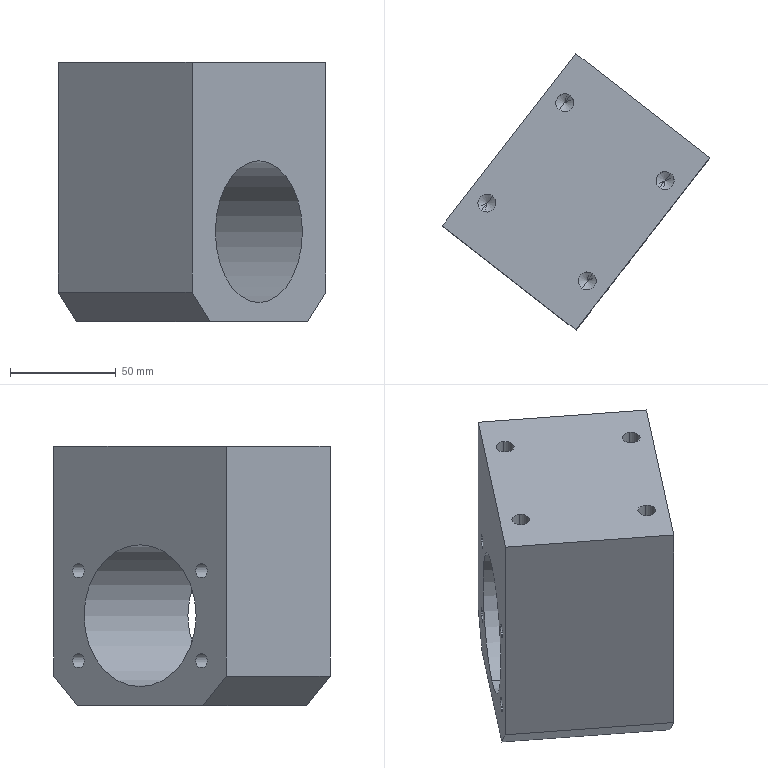Component | SolidWorks | 0803_206_Holder-1 | 1 solid | 42 faces | box 126.35 x 130.42 x 122.5 mm | volume 700208 mm3 | cylinder 18 | cone 16 | plane 8 | commonest cylinder face diameters 8.5 x8 6.8 x8 67 x2
STEP:
#1=COLOUR_RGB('',0.7922,0.8196,0.9333);
#2=FILL_AREA_STYLE_COLOUR('',#1);
#3=FILL_AREA_STYLE('',(#2));
#4=SURFACE_STYLE_FILL_AREA(#3);
#5=SURFACE_SIDE_STYLE('',(#4));
#6=SURFACE_STYLE_USAGE(.BOTH.,#5);
#7=PRESENTATION_STYLE_ASSIGNMENT((#6));
#8=CARTESIAN_POINT('',(2.329,25.802,12.851));
#9=VERTEX_POINT('',#8);
#10=CARTESIAN_POINT('',(2.534,26.066,12.851));
#11=VERTEX_POINT('',#10);
#12=CARTESIAN_POINT('',(2.431,25.934,12.851));
#13=DIRECTION('',(-0.,-0.,1.));
#14=DIRECTION('',(0.6132,0.7899,0.));
#15=AXIS2_PLACEMENT_3D('',#12,#13,#14);
#16=CIRCLE('',#15,0.1673);
#17=EDGE_CURVE('',#9,#11,#16,.T.);
#18=ORIENTED_EDGE('',*,*,#17,.F.);
#19=CARTESIAN_POINT('',(2.329,25.802,14.032));
#20=VERTEX_POINT('',#19);
#21=CARTESIAN_POINT('',(2.329,25.802,14.032));
#22=DIRECTION('',(-0.,-0.,1.));
#23=VECTOR('',#22,39.37);
#24=LINE('',#21,#23);
#25=EDGE_CURVE('',#9,#20,#24,.T.);
#26=ORIENTED_EDGE('',*,*,#25,.T.);
#27=CARTESIAN_POINT('',(2.534,26.066,14.032));
#28=VERTEX_POINT('',#27);
#29=CARTESIAN_POINT('',(2.431,25.934,14.032));
#30=DIRECTION('',(-0.,-0.,1.));
#31=DIRECTION('',(0.6132,0.7899,0.));
#32=AXIS2_PLACEMENT_3D('',#29,#30,#31);
#33=CIRCLE('',#32,0.1673);
#34=EDGE_CURVE('',#20,#28,#33,.T.);
#35=ORIENTED_EDGE('',*,*,#34,.T.);
#36=CARTESIAN_POINT('',(2.534,26.066,14.032));
#37=DIRECTION('',(-0.,-0.,1.));
#38=VECTOR('',#37,39.37);
#39=LINE('',#36,#38);
#40=EDGE_CURVE('',#11,#28,#39,.T.);
#41=ORIENTED_EDGE('',*,*,#40,.F.);
#42=EDGE_LOOP('',(#18,#26,#35,#41));
#43=FACE_OUTER_BOUND('',#42,.T.);
#44=CARTESIAN_POINT('',(2.431,25.934,14.032));
#45=DIRECTION('',(-0.,-0.,1.));
#46=DIRECTION('',(0.6132,0.7899,0.));
#47=AXIS2_PLACEMENT_3D('',#44,#45,#46);
#48=CYLINDRICAL_SURFACE('',#47,0.1673);
#49=ADVANCED_FACE('',(#43),#48,.F.);
#50=CARTESIAN_POINT('',(2.431,25.934,12.75));
#51=VERTEX_POINT('',#50);
#52=CARTESIAN_POINT('',(2.534,26.066,12.851));
#53=DIRECTION('',(0.5256,0.6771,0.515));
#54=VECTOR('',#53,39.37);
#55=LINE('',#52,#54);
#56=EDGE_CURVE('',#51,#11,#55,.T.);
#57=ORIENTED_EDGE('',*,*,#56,.F.);
#58=CARTESIAN_POINT('',(2.329,25.802,12.851));
#59=DIRECTION('',(-0.5256,-0.6771,0.515));
#60=VECTOR('',#59,39.37);
#61=LINE('',#58,#60);
#62=EDGE_CURVE('',#51,#9,#61,.T.);
#63=ORIENTED_EDGE('',*,*,#62,.T.);
#64=ORIENTED_EDGE('',*,*,#17,.T.);
#65=EDGE_LOOP('',(#57,#63,#64));
#66=FACE_OUTER_BOUND('',#65,.T.);
#67=CARTESIAN_POINT('',(2.431,25.934,12.851));
#68=DIRECTION('',(-0.,-0.,1.));
#69=DIRECTION('',(0.6132,0.7899,0.));
#70=AXIS2_PLACEMENT_3D('',#67,#68,#69);
#71=CONICAL_SURFACE('',#70,0.1673,1.03);
#72=ADVANCED_FACE('',(#66),#71,.F.);
#73=CARTESIAN_POINT('',(4.195,24.353,12.851));
#74=VERTEX_POINT('',#73);
#75=CARTESIAN_POINT('',(4.4,24.618,12.851));
#76=VERTEX_POINT('',#75);
#77=CARTESIAN_POINT('',(4.297,24.486,12.851));
#78=DIRECTION('',(-0.,-0.,1.));
#79=DIRECTION('',(0.6132,0.7899,0.));
#80=AXIS2_PLACEMENT_3D('',#77,#78,#79);
#81=CIRCLE('',#80,0.1673);
#82=EDGE_CURVE('',#74,#76,#81,.T.);
#83=ORIENTED_EDGE('',*,*,#82,.F.);
#84=CARTESIAN_POINT('',(4.195,24.353,14.032));
#85=VERTEX_POINT('',#84);
#86=CARTESIAN_POINT('',(4.195,24.353,14.032));
#87=DIRECTION('',(-0.,-0.,1.));
#88=VECTOR('',#87,39.37);
#89=LINE('',#86,#88);
#90=EDGE_CURVE('',#74,#85,#89,.T.);
#91=ORIENTED_EDGE('',*,*,#90,.T.);
#92=CARTESIAN_POINT('',(4.4,24.618,14.032));
#93=VERTEX_POINT('',#92);
#94=CARTESIAN_POINT('',(4.297,24.486,14.032));
#95=DIRECTION('',(-0.,-0.,1.));
#96=DIRECTION('',(0.6132,0.7899,0.));
#97=AXIS2_PLACEMENT_3D('',#94,#95,#96);
#98=CIRCLE('',#97,0.1673);
#99=EDGE_CURVE('',#85,#93,#98,.T.);
#100=ORIENTED_EDGE('',*,*,#99,.T.);
#101=CARTESIAN_POINT('',(4.4,24.618,14.032));
#102=DIRECTION('',(-0.,-0.,1.));
#103=VECTOR('',#102,39.37);
#104=LINE('',#101,#103);
#105=EDGE_CURVE('',#76,#93,#104,.T.);
#106=ORIENTED_EDGE('',*,*,#105,.F.);
#107=EDGE_LOOP('',(#83,#91,#100,#106));
#108=FACE_OUTER_BOUND('',#107,.T.);
#109=CARTESIAN_POINT('',(4.297,24.486,14.032));
#110=DIRECTION('',(-0.,-0.,1.));
#111=DIRECTION('',(0.6132,0.7899,0.));
#112=AXIS2_PLACEMENT_3D('',#109,#110,#111);
#113=CYLINDRICAL_SURFACE('',#112,0.1673);
#114=ADVANCED_FACE('',(#108),#113,.F.);
#115=CARTESIAN_POINT('',(4.297,24.486,12.75));
#116=VERTEX_POINT('',#115);
#117=CARTESIAN_POINT('',(4.4,24.618,12.851));
#118=DIRECTION('',(0.5256,0.6771,0.515));
#119=VECTOR('',#118,39.37);
#120=LINE('',#117,#119);
#121=EDGE_CURVE('',#116,#76,#120,.T.);
#122=ORIENTED_EDGE('',*,*,#121,.F.);
#123=CARTESIAN_POINT('',(4.195,24.353,12.851));
#124=DIRECTION('',(-0.5256,-0.6771,0.515));
#125=VECTOR('',#124,39.37);
#126=LINE('',#123,#125);
#127=EDGE_CURVE('',#116,#74,#126,.T.);
#128=ORIENTED_EDGE('',*,*,#127,.T.);
#129=ORIENTED_EDGE('',*,*,#82,.T.);
#130=EDGE_LOOP('',(#122,#128,#129));
#131=FACE_OUTER_BOUND('',#130,.T.);
#132=CARTESIAN_POINT('',(4.297,24.486,12.851));
#133=DIRECTION('',(-0.,-0.,1.));
#134=DIRECTION('',(0.6132,0.7899,0.));
#135=AXIS2_PLACEMENT_3D('',#132,#133,#134);
#136=CONICAL_SURFACE('',#135,0.1673,1.03);
#137=ADVANCED_FACE('',(#131),#136,.F.);
#138=CARTESIAN_POINT('',(5.643,26.219,12.851));
#139=VERTEX_POINT('',#138);
#140=CARTESIAN_POINT('',(5.848,26.484,12.851));
#141=VERTEX_POINT('',#140);
#142=CARTESIAN_POINT('',(5.746,26.352,12.851));
#143=DIRECTION('',(-0.,-0.,1.));
#144=DIRECTION('',(0.6132,0.7899,0.));
#145=AXIS2_PLACEMENT_3D('',#142,#143,#144);
#146=CIRCLE('',#145,0.1673);
#147=EDGE_CURVE('',#139,#141,#146,.T.);
#148=ORIENTED_EDGE('',*,*,#147,.F.);
#149=CARTESIAN_POINT('',(5.643,26.219,14.032));
#150=VERTEX_POINT('',#149);
#151=CARTESIAN_POINT('',(5.643,26.219,14.032));
#152=DIRECTION('',(-0.,-0.,1.));
#153=VECTOR('',#152,39.37);
#154=LINE('',#151,#153);
#155=EDGE_CURVE('',#139,#150,#154,.T.);
#156=ORIENTED_EDGE('',*,*,#155,.T.);
#157=CARTESIAN_POINT('',(5.848,26.484,14.032));
#158=VERTEX_POINT('',#157);
#159=CARTESIAN_POINT('',(5.746,26.352,14.032));
#160=DIRECTION('',(-0.,-0.,1.));
#161=DIRECTION('',(0.6132,0.7899,0.));
#162=AXIS2_PLACEMENT_3D('',#159,#160,#161);
#163=CIRCLE('',#162,0.1673);
#164=EDGE_CURVE('',#150,#158,#163,.T.);
#165=ORIENTED_EDGE('',*,*,#164,.T.);
#166=CARTESIAN_POINT('',(5.848,26.484,14.032));
#167=DIRECTION('',(-0.,-0.,1.));
#168=VECTOR('',#167,39.37);
#169=LINE('',#166,#168);
#170=EDGE_CURVE('',#141,#158,#169,.T.);
#171=ORIENTED_EDGE('',*,*,#170,.F.);
#172=EDGE_LOOP('',(#148,#156,#165,#171));
#173=FACE_OUTER_BOUND('',#172,.T.);
#174=CARTESIAN_POINT('',(5.746,26.352,14.032));
#175=DIRECTION('',(-0.,-0.,1.));
#176=DIRECTION('',(0.6132,0.7899,0.));
#177=AXIS2_PLACEMENT_3D('',#174,#175,#176);
#178=CYLINDRICAL_SURFACE('',#177,0.1673);
#179=ADVANCED_FACE('',(#173),#178,.F.);
#180=CARTESIAN_POINT('',(5.746,26.352,12.75));
#181=VERTEX_POINT('',#180);
#182=CARTESIAN_POINT('',(5.848,26.484,12.851));
#183=DIRECTION('',(0.5256,0.6771,0.515));
#184=VECTOR('',#183,39.37);
#185=LINE('',#182,#184);
#186=EDGE_CURVE('',#181,#141,#185,.T.);
#187=ORIENTED_EDGE('',*,*,#186,.F.);
#188=CARTESIAN_POINT('',(5.643,26.219,12.851));
#189=DIRECTION('',(-0.5256,-0.6771,0.515));
#190=VECTOR('',#189,39.37);
#191=LINE('',#188,#190);
#192=EDGE_CURVE('',#181,#139,#191,.T.);
#193=ORIENTED_EDGE('',*,*,#192,.T.);
#194=ORIENTED_EDGE('',*,*,#147,.T.);
#195=EDGE_LOOP('',(#187,#193,#194));
#196=FACE_OUTER_BOUND('',#195,.T.);
#197=CARTESIAN_POINT('',(5.746,26.352,12.851));
#198=DIRECTION('',(-0.,-0.,1.));
#199=DIRECTION('',(0.6132,0.7899,0.));
#200=AXIS2_PLACEMENT_3D('',#197,#198,#199);
#201=CONICAL_SURFACE('',#200,0.1673,1.03);
#202=ADVANCED_FACE('',(#196),#201,.F.);
#203=CARTESIAN_POINT('',(3.777,27.668,12.851));
#204=VERTEX_POINT('',#203);
#205=CARTESIAN_POINT('',(3.982,27.932,12.851));
#206=VERTEX_POINT('',#205);
#207=CARTESIAN_POINT('',(3.88,27.8,12.851));
#208=DIRECTION('',(-0.,-0.,1.));
#209=DIRECTION('',(0.6132,0.7899,0.));
#210=AXIS2_PLACEMENT_3D('',#207,#208,#209);
#211=CIRCLE('',#210,0.1673);
#212=EDGE_CURVE('',#204,#206,#211,.T.);
#213=ORIENTED_EDGE('',*,*,#212,.F.);
#214=CARTESIAN_POINT('',(3.777,27.668,14.032));
#215=VERTEX_POINT('',#214);
#216=CARTESIAN_POINT('',(3.777,27.668,14.032));
#217=DIRECTION('',(-0.,-0.,1.));
#218=VECTOR('',#217,39.37);
#219=LINE('',#216,#218);
#220=EDGE_CURVE('',#204,#215,#219,.T.);
#221=ORIENTED_EDGE('',*,*,#220,.T.);
#222=CARTESIAN_POINT('',(3.982,27.932,14.032));
#223=VERTEX_POINT('',#222);
#224=CARTESIAN_POINT('',(3.88,27.8,14.032));
#225=DIRECTION('',(-0.,-0.,1.));
#226=DIRECTION('',(0.6132,0.7899,0.));
#227=AXIS2_PLACEMENT_3D('',#224,#225,#226);
#228=CIRCLE('',#227,0.1673);
#229=EDGE_CURVE('',#215,#223,#228,.T.);
#230=ORIENTED_EDGE('',*,*,#229,.T.);
#231=CARTESIAN_POINT('',(3.982,27.932,14.032));
#232=DIRECTION('',(-0.,-0.,1.));
#233=VECTOR('',#232,39.37);
#234=LINE('',#231,#233);
#235=EDGE_CURVE('',#206,#223,#234,.T.);
#236=ORIENTED_EDGE('',*,*,#235,.F.);
#237=EDGE_LOOP('',(#213,#221,#230,#236));
#238=FACE_OUTER_BOUND('',#237,.T.);
#239=CARTESIAN_POINT('',(3.88,27.8,14.032));
#240=DIRECTION('',(-0.,-0.,1.));
#241=DIRECTION('',(0.6132,0.7899,0.));
#242=AXIS2_PLACEMENT_3D('',#239,#240,#241);
#243=CYLINDRICAL_SURFACE('',#242,0.1673);
#244=ADVANCED_FACE('',(#238),#243,.F.);
#245=CARTESIAN_POINT('',(3.88,27.8,12.75));
#246=VERTEX_POINT('',#245);
#247=CARTESIAN_POINT('',(3.982,27.932,12.851));
#248=DIRECTION('',(0.5256,0.6771,0.515));
#249=VECTOR('',#248,39.37);
#250=LINE('',#247,#249);
#251=EDGE_CURVE('',#246,#206,#250,.T.);
#252=ORIENTED_EDGE('',*,*,#251,.F.);
#253=CARTESIAN_POINT('',(3.777,27.668,12.851));
#254=DIRECTION('',(-0.5256,-0.6771,0.515));
#255=VECTOR('',#254,39.37);
#256=LINE('',#253,#255);
#257=EDGE_CURVE('',#246,#204,#256,.T.);
#258=ORIENTED_EDGE('',*,*,#257,.T.);
#259=ORIENTED_EDGE('',*,*,#212,.T.);
#260=EDGE_LOOP('',(#252,#258,#259));
#261=FACE_OUTER_BOUND('',#260,.T.);
#262=CARTESIAN_POINT('',(3.88,27.8,12.851));
#263=DIRECTION('',(-0.,-0.,1.));
#264=DIRECTION('',(0.6132,0.7899,0.));
#265=AXIS2_PLACEMENT_3D('',#262,#263,#264);
#266=CONICAL_SURFACE('',#265,0.1673,1.03);
#267=ADVANCED_FACE('',(#261),#266,.F.);
#268=CARTESIAN_POINT('',(4.666,27.529,11.585));
#269=VERTEX_POINT('',#268);
#270=CARTESIAN_POINT('',(4.666,27.529,11.853));
#271=VERTEX_POINT('',#270);
#272=CARTESIAN_POINT('',(4.666,27.529,11.719));
#273=DIRECTION('',(-0.7899,0.6132,0.));
#274=DIRECTION('',(0.,0.,1.));
#275=AXIS2_PLACEMENT_3D('',#272,#273,#274);
#276=CIRCLE('',#275,0.1339);
#277=EDGE_CURVE('',#269,#271,#276,.T.);
#278=ORIENTED_EDGE('',*,*,#277,.F.);
#279=CARTESIAN_POINT('',(3.733,28.253,11.585));
#280=VERTEX_POINT('',#279);
#281=CARTESIAN_POINT('',(3.733,28.253,11.585));
#282=DIRECTION('',(-0.7899,0.6132,0.));
#283=VECTOR('',#282,39.37);
#284=LINE('',#281,#283);
#285=EDGE_CURVE('',#269,#280,#284,.T.);
#286=ORIENTED_EDGE('',*,*,#285,.T.);
#287=CARTESIAN_POINT('',(3.733,28.253,11.853));
#288=VERTEX_POINT('',#287);
#289=CARTESIAN_POINT('',(3.733,28.253,11.719));
#290=DIRECTION('',(-0.7899,0.6132,0.));
#291=DIRECTION('',(0.,0.,1.));
#292=AXIS2_PLACEMENT_3D('',#289,#290,#291);
#293=CIRCLE('',#292,0.1339);
#294=EDGE_CURVE('',#280,#288,#293,.T.);
#295=ORIENTED_EDGE('',*,*,#294,.T.);
#296=CARTESIAN_POINT('',(3.733,28.253,11.853));
#297=DIRECTION('',(-0.7899,0.6132,0.));
#298=VECTOR('',#297,39.37);
#299=LINE('',#296,#298);
#300=EDGE_CURVE('',#271,#288,#299,.T.);
#301=ORIENTED_EDGE('',*,*,#300,.F.);
#302=EDGE_LOOP('',(#278,#286,#295,#301));
#303=FACE_OUTER_BOUND('',#302,.T.);
#304=CARTESIAN_POINT('',(3.733,28.253,11.719));
#305=DIRECTION('',(-0.7899,0.6132,0.));
#306=DIRECTION('',(0.,0.,1.));
#307=AXIS2_PLACEMENT_3D('',#304,#305,#306);
#308=CYLINDRICAL_SURFACE('',#307,0.1339);
#309=ADVANCED_FACE('',(#303),#308,.F.);
#310=CARTESIAN_POINT('',(4.73,27.48,11.719));
#311=VERTEX_POINT('',#310);
#312=CARTESIAN_POINT('',(4.666,27.529,11.853));
#313=DIRECTION('',(-0.4068,0.3158,0.8572));
#314=VECTOR('',#313,39.37);
#315=LINE('',#312,#314);
#316=EDGE_CURVE('',#311,#271,#315,.T.);
#317=ORIENTED_EDGE('',*,*,#316,.F.);
#318=CARTESIAN_POINT('',(4.666,27.529,11.585));
#319=DIRECTION('',(-0.4068,0.3158,-0.8572));
#320=VECTOR('',#319,39.37);
#321=LINE('',#318,#320);
#322=EDGE_CURVE('',#311,#269,#321,.T.);
#323=ORIENTED_EDGE('',*,*,#322,.T.);
#324=ORIENTED_EDGE('',*,*,#277,.T.);
#325=EDGE_LOOP('',(#317,#323,#324));
#326=FACE_OUTER_BOUND('',#325,.T.);
#327=CARTESIAN_POINT('',(4.666,27.529,11.719));
#328=DIRECTION('',(-0.7899,0.6132,0.));
#329=DIRECTION('',(0.,0.,1.));
#330=AXIS2_PLACEMENT_3D('',#327,#328,#329);
#331=CONICAL_SURFACE('',#330,0.1339,1.03);
#332=ADVANCED_FACE('',(#326),#331,.F.);
#333=CARTESIAN_POINT('',(4.666,27.529,9.912));
#334=VERTEX_POINT('',#333);
#335=CARTESIAN_POINT('',(4.666,27.529,10.18));
#336=VERTEX_POINT('',#335);
#337=CARTESIAN_POINT('',(4.666,27.529,10.046));
#338=DIRECTION('',(-0.7899,0.6132,0.));
#339=DIRECTION('',(0.,0.,1.));
#340=AXIS2_PLACEMENT_3D('',#337,#338,#339);
#341=CIRCLE('',#340,0.1339);
#342=EDGE_CURVE('',#334,#336,#341,.T.);
#343=ORIENTED_EDGE('',*,*,#342,.F.);
#344=CARTESIAN_POINT('',(3.733,28.253,9.912));
#345=VERTEX_POINT('',#344);
#346=CARTESIAN_POINT('',(3.733,28.253,9.912));
#347=DIRECTION('',(-0.7899,0.6132,0.));
#348=VECTOR('',#347,39.37);
#349=LINE('',#346,#348);
#350=EDGE_CURVE('',#334,#345,#349,.T.);
#351=ORIENTED_EDGE('',*,*,#350,.T.);
#352=CARTESIAN_POINT('',(3.733,28.253,10.18));
#353=VERTEX_POINT('',#352);
#354=CARTESIAN_POINT('',(3.733,28.253,10.046));
#355=DIRECTION('',(-0.7899,0.6132,0.));
#356=DIRECTION('',(0.,0.,1.));
#357=AXIS2_PLACEMENT_3D('',#354,#355,#356);
#358=CIRCLE('',#357,0.1339);
#359=EDGE_CURVE('',#345,#353,#358,.T.);
#360=ORIENTED_EDGE('',*,*,#359,.T.);
#361=CARTESIAN_POINT('',(3.733,28.253,10.18));
#362=DIRECTION('',(-0.7899,0.6132,0.));
#363=VECTOR('',#362,39.37);
#364=LINE('',#361,#363);
#365=EDGE_CURVE('',#336,#353,#364,.T.);
#366=ORIENTED_EDGE('',*,*,#365,.F.);
#367=EDGE_LOOP('',(#343,#351,#360,#366));
#368=FACE_OUTER_BOUND('',#367,.T.);
#369=CARTESIAN_POINT('',(3.733,28.253,10.046));
#370=DIRECTION('',(-0.7899,0.6132,0.));
#371=DIRECTION('',(0.,0.,1.));
#372=AXIS2_PLACEMENT_3D('',#369,#370,#371);
#373=CYLINDRICAL_SURFACE('',#372,0.1339);
#374=ADVANCED_FACE('',(#368),#373,.F.);
#375=CARTESIAN_POINT('',(4.73,27.48,10.046));
#376=VERTEX_POINT('',#375);
#377=CARTESIAN_POINT('',(4.666,27.529,10.18));
#378=DIRECTION('',(-0.4068,0.3158,0.8572));
#379=VECTOR('',#378,39.37);
#380=LINE('',#377,#379);
#381=EDGE_CURVE('',#376,#336,#380,.T.);
#382=ORIENTED_EDGE('',*,*,#381,.F.);
#383=CARTESIAN_POINT('',(4.666,27.529,9.912));
#384=DIRECTION('',(-0.4068,0.3158,-0.8572));
#385=VECTOR('',#384,39.37);
#386=LINE('',#383,#385);
#387=EDGE_CURVE('',#376,#334,#386,.T.);
#388=ORIENTED_EDGE('',*,*,#387,.T.);
#389=ORIENTED_EDGE('',*,*,#342,.T.);
#390=EDGE_LOOP('',(#382,#388,#389));
#391=FACE_OUTER_BOUND('',#390,.T.);
#392=CARTESIAN_POINT('',(4.666,27.529,10.046));
#393=DIRECTION('',(-0.7899,0.6132,0.));
#394=DIRECTION('',(0.,0.,1.));
#395=AXIS2_PLACEMENT_3D('',#392,#393,#394);
#396=CONICAL_SURFACE('',#395,0.1339,1.03);
#397=ADVANCED_FACE('',(#391),#396,.F.);
#398=CARTESIAN_POINT('',(2.889,25.24,9.912));
#399=VERTEX_POINT('',#398);
#400=CARTESIAN_POINT('',(2.889,25.24,10.18));
#401=VERTEX_POINT('',#400);
#402=CARTESIAN_POINT('',(2.889,25.24,10.046));
#403=DIRECTION('',(-0.7899,0.6132,0.));
#404=DIRECTION('',(0.,0.,1.));
#405=AXIS2_PLACEMENT_3D('',#402,#403,#404);
#406=CIRCLE('',#405,0.1339);
#407=EDGE_CURVE('',#399,#401,#406,.T.);
#408=ORIENTED_EDGE('',*,*,#407,.F.);
#409=CARTESIAN_POINT('',(1.956,25.964,9.912));
#410=VERTEX_POINT('',#409);
#411=CARTESIAN_POINT('',(1.956,25.964,9.912));
#412=DIRECTION('',(-0.7899,0.6132,0.));
#413=VECTOR('',#412,39.37);
#414=LINE('',#411,#413);
#415=EDGE_CURVE('',#399,#410,#414,.T.);
#416=ORIENTED_EDGE('',*,*,#415,.T.);
#417=CARTESIAN_POINT('',(1.956,25.964,10.18));
#418=VERTEX_POINT('',#417);
#419=CARTESIAN_POINT('',(1.956,25.964,10.046));
#420=DIRECTION('',(-0.7899,0.6132,0.));
#421=DIRECTION('',(-0.,0.,1.));
#422=AXIS2_PLACEMENT_3D('',#419,#420,#421);
#423=CIRCLE('',#422,0.1339);
#424=EDGE_CURVE('',#410,#418,#423,.T.);
#425=ORIENTED_EDGE('',*,*,#424,.T.);
#426=CARTESIAN_POINT('',(1.956,25.964,10.18));
#427=DIRECTION('',(-0.7899,0.6132,0.));
#428=VECTOR('',#427,39.37);
#429=LINE('',#426,#428);
#430=EDGE_CURVE('',#401,#418,#429,.T.);
#431=ORIENTED_EDGE('',*,*,#430,.F.);
#432=EDGE_LOOP('',(#408,#416,#425,#431));
#433=FACE_OUTER_BOUND('',#432,.T.);
#434=CARTESIAN_POINT('',(1.956,25.964,10.046));
#435=DIRECTION('',(-0.7899,0.6132,0.));
#436=DIRECTION('',(-0.,0.,1.));
#437=AXIS2_PLACEMENT_3D('',#434,#435,#436);
#438=CYLINDRICAL_SURFACE('',#437,0.1339);
#439=ADVANCED_FACE('',(#433),#438,.F.);
#440=CARTESIAN_POINT('',(2.952,25.19,10.046));
#441=VERTEX_POINT('',#440);
#442=CARTESIAN_POINT('',(2.889,25.24,10.18));
#443=DIRECTION('',(-0.4068,0.3158,0.8572));
#444=VECTOR('',#443,39.37);
#445=LINE('',#442,#444);
#446=EDGE_CURVE('',#441,#401,#445,.T.);
#447=ORIENTED_EDGE('',*,*,#446,.F.);
#448=CARTESIAN_POINT('',(2.889,25.24,9.912));
#449=DIRECTION('',(-0.4068,0.3158,-0.8572));
#450=VECTOR('',#449,39.37);
#451=LINE('',#448,#450);
#452=EDGE_CURVE('',#441,#399,#451,.T.);
#453=ORIENTED_EDGE('',*,*,#452,.T.);
#454=ORIENTED_EDGE('',*,*,#407,.T.);
#455=EDGE_LOOP('',(#447,#453,#454));
#456=FACE_OUTER_BOUND('',#455,.T.);
#457=CARTESIAN_POINT('',(2.889,25.24,10.046));
#458=DIRECTION('',(-0.7899,0.6132,0.));
#459=DIRECTION('',(0.,0.,1.));
#460=AXIS2_PLACEMENT_3D('',#457,#458,#459);
#461=CONICAL_SURFACE('',#460,0.1339,1.03);
#462=ADVANCED_FACE('',(#456),#461,.F.);
#463=CARTESIAN_POINT('',(2.889,25.24,11.585));
#464=VERTEX_POINT('',#463);
#465=CARTESIAN_POINT('',(2.889,25.24,11.853));
#466=VERTEX_POINT('',#465);
#467=CARTESIAN_POINT('',(2.889,25.24,11.719));
#468=DIRECTION('',(-0.7899,0.6132,0.));
#469=DIRECTION('',(0.,0.,1.));
#470=AXIS2_PLACEMENT_3D('',#467,#468,#469);
#471=CIRCLE('',#470,0.1339);
#472=EDGE_CURVE('',#464,#466,#471,.T.);
#473=ORIENTED_EDGE('',*,*,#472,.F.);
#474=CARTESIAN_POINT('',(1.956,25.964,11.585));
#475=VERTEX_POINT('',#474);
#476=CARTESIAN_POINT('',(1.956,25.964,11.585));
#477=DIRECTION('',(-0.7899,0.6132,0.));
#478=VECTOR('',#477,39.37);
#479=LINE('',#476,#478);
#480=EDGE_CURVE('',#464,#475,#479,.T.);
#481=ORIENTED_EDGE('',*,*,#480,.T.);
#482=CARTESIAN_POINT('',(1.956,25.964,11.853));
#483=VERTEX_POINT('',#482);
#484=CARTESIAN_POINT('',(1.956,25.964,11.719));
#485=DIRECTION('',(-0.7899,0.6132,0.));
#486=DIRECTION('',(-0.,0.,1.));
#487=AXIS2_PLACEMENT_3D('',#484,#485,#486);
#488=CIRCLE('',#487,0.1339);
#489=EDGE_CURVE('',#475,#483,#488,.T.);
#490=ORIENTED_EDGE('',*,*,#489,.T.);
#491=CARTESIAN_POINT('',(1.956,25.964,11.853));
#492=DIRECTION('',(-0.7899,0.6132,0.));
#493=VECTOR('',#492,39.37);
#494=LINE('',#491,#493);
#495=EDGE_CURVE('',#466,#483,#494,.T.);
#496=ORIENTED_EDGE('',*,*,#495,.F.);
#497=EDGE_LOOP('',(#473,#481,#490,#496));
#498=FACE_OUTER_BOUND('',#497,.T.);
#499=CARTESIAN_POINT('',(1.956,25.964,11.719));
#500=DIRECTION('',(-0.7899,0.6132,0.));
#501=DIRECTION('',(-0.,0.,1.));
#502=AXIS2_PLACEMENT_3D('',#499,#500,#501);
#503=CYLINDRICAL_SURFACE('',#502,0.1339);
#504=ADVANCED_FACE('',(#498),#503,.F.);
#505=CARTESIAN_POINT('',(2.952,25.19,11.719));
#506=VERTEX_POINT('',#505);
#507=CARTESIAN_POINT('',(2.889,25.24,11.853));
#508=DIRECTION('',(-0.4068,0.3158,0.8572));
#509=VECTOR('',#508,39.37);
#510=LINE('',#507,#509);
#511=EDGE_CURVE('',#506,#466,#510,.T.);
#512=ORIENTED_EDGE('',*,*,#511,.F.);
#513=CARTESIAN_POINT('',(2.889,25.24,11.585));
#514=DIRECTION('',(-0.4068,0.3158,-0.8572));
#515=VECTOR('',#514,39.37);
#516=LINE('',#513,#515);
#517=EDGE_CURVE('',#506,#464,#516,.T.);
#518=ORIENTED_EDGE('',*,*,#517,.T.);
#519=ORIENTED_EDGE('',*,*,#472,.T.);
#520=EDGE_LOOP('',(#512,#518,#519));
#521=FACE_OUTER_BOUND('',#520,.T.);
#522=CARTESIAN_POINT('',(2.889,25.24,11.719));
#523=DIRECTION('',(-0.7899,0.6132,0.));
#524=DIRECTION('',(0.,0.,1.));
#525=AXIS2_PLACEMENT_3D('',#522,#523,#524);
#526=CONICAL_SURFACE('',#525,0.1339,1.03);
#527=ADVANCED_FACE('',(#521),#526,.F.);
#528=CARTESIAN_POINT('',(5.332,25.177,9.563));
#529=VERTEX_POINT('',#528);
#530=CARTESIAN_POINT('',(5.332,25.177,12.201));
#531=VERTEX_POINT('',#530);
#532=CARTESIAN_POINT('',(5.332,25.177,10.882));
#533=DIRECTION('',(-0.7899,0.6132,0.));
#534=DIRECTION('',(-0.,-0.,1.));
#535=AXIS2_PLACEMENT_3D('',#532,#533,#534);
#536=CIRCLE('',#535,1.319);
#537=EDGE_CURVE('',#529,#531,#536,.T.);
#538=ORIENTED_EDGE('',*,*,#537,.F.);
#539=CARTESIAN_POINT('',(2.844,27.108,9.563));
#540=VERTEX_POINT('',#539);
#541=CARTESIAN_POINT('',(5.332,25.177,9.563));
#542=DIRECTION('',(-0.7899,0.6132,0.));
#543=VECTOR('',#542,39.37);
#544=LINE('',#541,#543);
#545=EDGE_CURVE('',#529,#540,#544,.T.);
#546=ORIENTED_EDGE('',*,*,#545,.T.);
#547=CARTESIAN_POINT('',(2.844,27.108,12.201));
#548=VERTEX_POINT('',#547);
#549=CARTESIAN_POINT('',(2.844,27.108,10.882));
#550=DIRECTION('',(-0.7899,0.6132,0.));
#551=DIRECTION('',(-0.,-0.,1.));
#552=AXIS2_PLACEMENT_3D('',#549,#550,#551);
#553=CIRCLE('',#552,1.319);
#554=EDGE_CURVE('',#540,#548,#553,.T.);
#555=ORIENTED_EDGE('',*,*,#554,.T.);
#556=CARTESIAN_POINT('',(5.332,25.177,12.201));
#557=DIRECTION('',(-0.7899,0.6132,0.));
#558=VECTOR('',#557,39.37);
#559=LINE('',#556,#558);
#560=EDGE_CURVE('',#531,#548,#559,.T.);
#561=ORIENTED_EDGE('',*,*,#560,.F.);
#562=EDGE_LOOP('',(#538,#546,#555,#561));
#563=FACE_OUTER_BOUND('',#562,.T.);
#564=CARTESIAN_POINT('',(5.332,25.177,10.882));
#565=DIRECTION('',(-0.7899,0.6132,0.));
#566=DIRECTION('',(-0.,-0.,1.));
#567=AXIS2_PLACEMENT_3D('',#564,#565,#566);
#568=CYLINDRICAL_SURFACE('',#567,1.319);
#569=ADVANCED_FACE('',(#563),#568,.F.);
#570=CARTESIAN_POINT('',(1.601,25.507,9.76));
#571=VERTEX_POINT('',#570);
#572=CARTESIAN_POINT('',(1.601,25.507,14.032));
#573=VERTEX_POINT('',#572);
#574=CARTESIAN_POINT('',(1.601,25.507,14.032));
#575=DIRECTION('',(-0.,-0.,1.));
#576=VECTOR('',#575,39.37);
#577=LINE('',#574,#576);
#578=EDGE_CURVE('',#571,#573,#577,.T.);
#579=ORIENTED_EDGE('',*,*,#578,.F.);
#580=CARTESIAN_POINT('',(4.089,23.576,9.76));
#581=VERTEX_POINT('',#580);
#582=CARTESIAN_POINT('',(1.601,25.507,9.76));
#583=DIRECTION('',(0.7899,-0.6132,-0.));
#584=VECTOR('',#583,39.37);
#585=LINE('',#582,#584);
#586=EDGE_CURVE('',#571,#581,#585,.T.);
#587=ORIENTED_EDGE('',*,*,#586,.T.);
#588=CARTESIAN_POINT('',(4.089,23.576,14.032));
#589=VERTEX_POINT('',#588);
#590=CARTESIAN_POINT('',(4.089,23.576,14.032));
#591=DIRECTION('',(-0.,-0.,1.));
#592=VECTOR('',#591,39.37);
#593=LINE('',#590,#592);
#594=EDGE_CURVE('',#581,#589,#593,.T.);
#595=ORIENTED_EDGE('',*,*,#594,.T.);
#596=CARTESIAN_POINT('',(1.601,25.507,14.032));
#597=DIRECTION('',(0.7899,-0.6132,-0.));
#598=VECTOR('',#597,39.37);
#599=LINE('',#596,#598);
#600=EDGE_CURVE('',#573,#589,#599,.T.);
#601=ORIENTED_EDGE('',*,*,#600,.F.);
#602=EDGE_LOOP('',(#579,#587,#595,#601));
#603=FACE_OUTER_BOUND('',#602,.T.);
#604=CARTESIAN_POINT('',(1.601,25.507,14.032));
#605=DIRECTION('',(0.6132,0.7899,0.));
#606=DIRECTION('',(0.,0.,-1.));
#607=AXIS2_PLACEMENT_3D('',#604,#605,#606);
#608=PLANE('',#607);
#609=ADVANCED_FACE('',(#603),#608,.F.);
#610=CARTESIAN_POINT('',(2.431,25.934,14.032));
#611=DIRECTION('',(-0.,-0.,1.));
#612=DIRECTION('',(0.6132,0.7899,0.));
#613=AXIS2_PLACEMENT_3D('',#610,#611,#612);
#614=CIRCLE('',#613,0.1673);
#615=EDGE_CURVE('',#28,#20,#614,.T.);
#616=ORIENTED_EDGE('',*,*,#615,.F.);
#617=ORIENTED_EDGE('',*,*,#34,.F.);
#618=EDGE_LOOP('',(#616,#617));
#619=FACE_BOUND('',#618,.T.);
#620=CARTESIAN_POINT('',(4.297,24.486,14.032));
#621=DIRECTION('',(-0.,-0.,1.));
#622=DIRECTION('',(0.6132,0.7899,0.));
#623=AXIS2_PLACEMENT_3D('',#620,#621,#622);
#624=CIRCLE('',#623,0.1673);
#625=EDGE_CURVE('',#93,#85,#624,.T.);
#626=ORIENTED_EDGE('',*,*,#625,.F.);
#627=ORIENTED_EDGE('',*,*,#99,.F.);
#628=EDGE_LOOP('',(#626,#627));
#629=FACE_BOUND('',#628,.T.);
#630=CARTESIAN_POINT('',(5.746,26.352,14.032));
#631=DIRECTION('',(-0.,-0.,1.));
#632=DIRECTION('',(0.6132,0.7899,0.));
#633=AXIS2_PLACEMENT_3D('',#630,#631,#632);
#634=CIRCLE('',#633,0.1673);
#635=EDGE_CURVE('',#158,#150,#634,.T.);
#636=ORIENTED_EDGE('',*,*,#635,.F.);
#637=ORIENTED_EDGE('',*,*,#164,.F.);
#638=EDGE_LOOP('',(#636,#637));
#639=FACE_BOUND('',#638,.T.);
#640=CARTESIAN_POINT('',(3.88,27.8,14.032));
#641=DIRECTION('',(-0.,-0.,1.));
#642=DIRECTION('',(0.6132,0.7899,0.));
#643=AXIS2_PLACEMENT_3D('',#640,#641,#642);
#644=CIRCLE('',#643,0.1673);
#645=EDGE_CURVE('',#223,#215,#644,.T.);
#646=ORIENTED_EDGE('',*,*,#645,.F.);
#647=ORIENTED_EDGE('',*,*,#229,.F.);
#648=EDGE_LOOP('',(#646,#647));
#649=FACE_BOUND('',#648,.T.);
#650=CARTESIAN_POINT('',(6.576,26.779,14.032));
#651=VERTEX_POINT('',#650);
#652=CARTESIAN_POINT('',(4.089,23.576,14.032));
#653=DIRECTION('',(0.6132,0.7899,0.));
#654=VECTOR('',#653,39.37);
#655=LINE('',#652,#654);
#656=EDGE_CURVE('',#589,#651,#655,.T.);
#657=ORIENTED_EDGE('',*,*,#656,.T.);
#658=CARTESIAN_POINT('',(4.088,28.71,14.032));
#659=VERTEX_POINT('',#658);
#660=CARTESIAN_POINT('',(4.088,28.71,14.032));
#661=DIRECTION('',(0.7899,-0.6132,-0.));
#662=VECTOR('',#661,39.37);
#663=LINE('',#660,#662);
#664=EDGE_CURVE('',#659,#651,#663,.T.);
#665=ORIENTED_EDGE('',*,*,#664,.F.);
#666=CARTESIAN_POINT('',(1.601,25.507,14.032));
#667=DIRECTION('',(0.6132,0.7899,0.));
#668=VECTOR('',#667,39.37);
#669=LINE('',#666,#668);
#670=EDGE_CURVE('',#573,#659,#669,.T.);
#671=ORIENTED_EDGE('',*,*,#670,.F.);
#672=ORIENTED_EDGE('',*,*,#600,.T.);
#673=EDGE_LOOP('',(#657,#665,#671,#672));
#674=FACE_OUTER_BOUND('',#673,.T.);
#675=CARTESIAN_POINT('',(1.601,25.507,14.032));
#676=DIRECTION('',(0.,0.,-1.));
#677=DIRECTION('',(-0.6132,-0.7899,-0.));
#678=AXIS2_PLACEMENT_3D('',#675,#676,#677);
#679=PLANE('',#678);
#680=ADVANCED_FACE('',(#619,#629,#639,#649,#674),#679,.F.);
#681=CARTESIAN_POINT('',(6.576,26.779,9.76));
#682=VERTEX_POINT('',#681);
#683=CARTESIAN_POINT('',(6.576,26.779,14.032));
#684=DIRECTION('',(0.,0.,-1.));
#685=VECTOR('',#684,39.37);
#686=LINE('',#683,#685);
#687=EDGE_CURVE('',#651,#682,#686,.T.);
#688=ORIENTED_EDGE('',*,*,#687,.T.);
#689=CARTESIAN_POINT('',(4.088,28.71,9.76));
#690=VERTEX_POINT('',#689);
#691=CARTESIAN_POINT('',(4.088,28.71,9.76));
#692=DIRECTION('',(-0.7899,0.6132,0.));
#693=VECTOR('',#692,39.37);
#694=LINE('',#691,#693);
#695=EDGE_CURVE('',#682,#690,#694,.T.);
#696=ORIENTED_EDGE('',*,*,#695,.T.);
#697=CARTESIAN_POINT('',(4.088,28.71,14.032));
#698=DIRECTION('',(0.,0.,-1.));
#699=VECTOR('',#698,39.37);
#700=LINE('',#697,#699);
#701=EDGE_CURVE('',#659,#690,#700,.T.);
#702=ORIENTED_EDGE('',*,*,#701,.F.);
#703=ORIENTED_EDGE('',*,*,#664,.T.);
#704=EDGE_LOOP('',(#688,#696,#702,#703));
#705=FACE_OUTER_BOUND('',#704,.T.);
#706=CARTESIAN_POINT('',(4.088,28.71,14.032));
#707=DIRECTION('',(-0.6132,-0.7899,-0.));
#708=DIRECTION('',(-0.,-0.,1.));
#709=AXIS2_PLACEMENT_3D('',#706,#707,#708);
#710=PLANE('',#709);
#711=ADVANCED_FACE('',(#705),#710,.F.);
#712=CARTESIAN_POINT('',(6.238,26.343,9.209));
#713=VERTEX_POINT('',#712);
#714=CARTESIAN_POINT('',(4.427,24.011,9.209));
#715=VERTEX_POINT('',#714);
#716=CARTESIAN_POINT('',(4.089,23.576,9.209));
#717=DIRECTION('',(-0.6132,-0.7899,-0.));
#718=VECTOR('',#717,39.37);
#719=LINE('',#716,#718);
#720=EDGE_CURVE('',#713,#715,#719,.T.);
#721=ORIENTED_EDGE('',*,*,#720,.T.);
#722=CARTESIAN_POINT('',(1.939,25.942,9.209));
#723=VERTEX_POINT('',#722);
#724=CARTESIAN_POINT('',(1.939,25.942,9.209));
#725=DIRECTION('',(-0.7899,0.6132,0.));
#726=VECTOR('',#725,39.37);
#727=LINE('',#724,#726);
#728=EDGE_CURVE('',#715,#723,#727,.T.);
#729=ORIENTED_EDGE('',*,*,#728,.T.);
#730=CARTESIAN_POINT('',(3.75,28.275,9.209));
#731=VERTEX_POINT('',#730);
#732=CARTESIAN_POINT('',(1.601,25.507,9.209));
#733=DIRECTION('',(-0.6132,-0.7899,-0.));
#734=VECTOR('',#733,39.37);
#735=LINE('',#732,#734);
#736=EDGE_CURVE('',#731,#723,#735,.T.);
#737=ORIENTED_EDGE('',*,*,#736,.F.);
#738=CARTESIAN_POINT('',(3.75,28.275,9.209));
#739=DIRECTION('',(0.7899,-0.6132,-0.));
#740=VECTOR('',#739,39.37);
#741=LINE('',#738,#740);
#742=EDGE_CURVE('',#731,#713,#741,.T.);
#743=ORIENTED_EDGE('',*,*,#742,.T.);
#744=EDGE_LOOP('',(#721,#729,#737,#743));
#745=FACE_OUTER_BOUND('',#744,.T.);
#746=CARTESIAN_POINT('',(1.601,25.507,9.209));
#747=DIRECTION('',(-0.,-0.,1.));
#748=DIRECTION('',(0.6132,0.7899,0.));
#749=AXIS2_PLACEMENT_3D('',#746,#747,#748);
#750=PLANE('',#749);
#751=ADVANCED_FACE('',(#745),#750,.F.);
#752=CARTESIAN_POINT('',(3.733,28.253,11.719));
#753=DIRECTION('',(-0.7899,0.6132,0.));
#754=DIRECTION('',(0.,0.,1.));
#755=AXIS2_PLACEMENT_3D('',#752,#753,#754);
#756=CIRCLE('',#755,0.1339);
#757=EDGE_CURVE('',#288,#280,#756,.T.);
#758=ORIENTED_EDGE('',*,*,#757,.F.);
#759=ORIENTED_EDGE('',*,*,#294,.F.);
#760=EDGE_LOOP('',(#758,#759));
#761=FACE_BOUND('',#760,.T.);
#762=CARTESIAN_POINT('',(3.733,28.253,10.046));
#763=DIRECTION('',(-0.7899,0.6132,0.));
#764=DIRECTION('',(0.,0.,1.));
#765=AXIS2_PLACEMENT_3D('',#762,#763,#764);
#766=CIRCLE('',#765,0.1339);
#767=EDGE_CURVE('',#353,#345,#766,.T.);
#768=ORIENTED_EDGE('',*,*,#767,.F.);
#769=ORIENTED_EDGE('',*,*,#359,.F.);
#770=EDGE_LOOP('',(#768,#769));
#771=FACE_BOUND('',#770,.T.);
#772=CARTESIAN_POINT('',(1.956,25.964,10.046));
#773=DIRECTION('',(-0.7899,0.6132,0.));
#774=DIRECTION('',(-0.,0.,1.));
#775=AXIS2_PLACEMENT_3D('',#772,#773,#774);
#776=CIRCLE('',#775,0.1339);
#777=EDGE_CURVE('',#418,#410,#776,.T.);
#778=ORIENTED_EDGE('',*,*,#777,.F.);
#779=ORIENTED_EDGE('',*,*,#424,.F.);
#780=EDGE_LOOP('',(#778,#779));
#781=FACE_BOUND('',#780,.T.);
#782=CARTESIAN_POINT('',(1.956,25.964,11.719));
#783=DIRECTION('',(-0.7899,0.6132,0.));
#784=DIRECTION('',(-0.,0.,1.));
#785=AXIS2_PLACEMENT_3D('',#782,#783,#784);
#786=CIRCLE('',#785,0.1339);
#787=EDGE_CURVE('',#483,#475,#786,.T.);
#788=ORIENTED_EDGE('',*,*,#787,.F.);
#789=ORIENTED_EDGE('',*,*,#489,.F.);
#790=EDGE_LOOP('',(#788,#789));
#791=FACE_BOUND('',#790,.T.);
#792=CARTESIAN_POINT('',(2.844,27.108,10.882));
#793=DIRECTION('',(-0.7899,0.6132,0.));
#794=DIRECTION('',(-0.,-0.,1.));
#795=AXIS2_PLACEMENT_3D('',#792,#793,#794);
#796=CIRCLE('',#795,1.319);
#797=EDGE_CURVE('',#548,#540,#796,.T.);
#798=ORIENTED_EDGE('',*,*,#797,.F.);
#799=ORIENTED_EDGE('',*,*,#554,.F.);
#800=EDGE_LOOP('',(#798,#799));
#801=FACE_BOUND('',#800,.T.);
#802=ORIENTED_EDGE('',*,*,#736,.T.);
#803=CARTESIAN_POINT('',(1.601,25.507,9.76));
#804=DIRECTION('',(-0.4336,-0.5586,0.7071));
#805=VECTOR('',#804,39.37);
#806=LINE('',#803,#805);
#807=EDGE_CURVE('',#723,#571,#806,.T.);
#808=ORIENTED_EDGE('',*,*,#807,.T.);
#809=ORIENTED_EDGE('',*,*,#578,.T.);
#810=ORIENTED_EDGE('',*,*,#670,.T.);
#811=ORIENTED_EDGE('',*,*,#701,.T.);
#812=CARTESIAN_POINT('',(3.75,28.275,9.209));
#813=DIRECTION('',(-0.4336,-0.5586,-0.7071));
#814=VECTOR('',#813,39.37);
#815=LINE('',#812,#814);
#816=EDGE_CURVE('',#690,#731,#815,.T.);
#817=ORIENTED_EDGE('',*,*,#816,.T.);
#818=EDGE_LOOP('',(#802,#808,#809,#810,#811,#817));
#819=FACE_OUTER_BOUND('',#818,.T.);
#820=CARTESIAN_POINT('',(1.601,25.507,9.209));
#821=DIRECTION('',(0.7899,-0.6132,-0.));
#822=DIRECTION('',(0.,0.,-1.));
#823=AXIS2_PLACEMENT_3D('',#820,#821,#822);
#824=PLANE('',#823);
#825=ADVANCED_FACE('',(#761,#771,#781,#791,#801,#819),#824,.F.);
#826=CARTESIAN_POINT('',(5.332,25.177,10.882));
#827=DIRECTION('',(-0.7899,0.6132,0.));
#828=DIRECTION('',(-0.,-0.,1.));
#829=AXIS2_PLACEMENT_3D('',#826,#827,#828);
#830=CIRCLE('',#829,1.319);
#831=EDGE_CURVE('',#531,#529,#830,.T.);
#832=ORIENTED_EDGE('',*,*,#831,.T.);
#833=ORIENTED_EDGE('',*,*,#537,.T.);
#834=EDGE_LOOP('',(#832,#833));
#835=FACE_BOUND('',#834,.T.);
#836=ORIENTED_EDGE('',*,*,#594,.F.);
#837=CARTESIAN_POINT('',(4.258,23.793,9.485));
#838=DIRECTION('',(0.4336,0.5586,-0.7071));
#839=VECTOR('',#838,39.37);
#840=LINE('',#837,#839);
#841=EDGE_CURVE('',#581,#715,#840,.T.);
#842=ORIENTED_EDGE('',*,*,#841,.T.);
#843=ORIENTED_EDGE('',*,*,#720,.F.);
#844=CARTESIAN_POINT('',(5.163,24.959,7.457));
#845=DIRECTION('',(0.4336,0.5586,0.7071));
#846=VECTOR('',#845,39.37);
#847=LINE('',#844,#846);
#848=EDGE_CURVE('',#713,#682,#847,.T.);
#849=ORIENTED_EDGE('',*,*,#848,.T.);
#850=ORIENTED_EDGE('',*,*,#687,.F.);
#851=ORIENTED_EDGE('',*,*,#656,.F.);
#852=EDGE_LOOP('',(#836,#842,#843,#849,#850,#851));
#853=FACE_OUTER_BOUND('',#852,.T.);
#854=CARTESIAN_POINT('',(4.089,23.576,9.209));
#855=DIRECTION('',(0.7899,-0.6132,-0.));
#856=DIRECTION('',(0.,0.,-1.));
#857=AXIS2_PLACEMENT_3D('',#854,#855,#856);
#858=PLANE('',#857);
#859=ADVANCED_FACE('',(#835,#853),#858,.T.);
#860=ORIENTED_EDGE('',*,*,#545,.F.);
#861=ORIENTED_EDGE('',*,*,#831,.F.);
#862=ORIENTED_EDGE('',*,*,#560,.T.);
#863=ORIENTED_EDGE('',*,*,#797,.T.);
#864=EDGE_LOOP('',(#860,#861,#862,#863));
#865=FACE_OUTER_BOUND('',#864,.T.);
#866=CARTESIAN_POINT('',(5.332,25.177,10.882));
#867=DIRECTION('',(-0.7899,0.6132,0.));
#868=DIRECTION('',(-0.,-0.,1.));
#869=AXIS2_PLACEMENT_3D('',#866,#867,#868);
#870=CYLINDRICAL_SURFACE('',#869,1.319);
#871=ADVANCED_FACE('',(#865),#870,.F.);
#872=ORIENTED_EDGE('',*,*,#517,.F.);
#873=ORIENTED_EDGE('',*,*,#511,.T.);
#874=CARTESIAN_POINT('',(2.889,25.24,11.719));
#875=DIRECTION('',(-0.7899,0.6132,0.));
#876=DIRECTION('',(0.,0.,1.));
#877=AXIS2_PLACEMENT_3D('',#874,#875,#876);
#878=CIRCLE('',#877,0.1339);
#879=EDGE_CURVE('',#466,#464,#878,.T.);
#880=ORIENTED_EDGE('',*,*,#879,.T.);
#881=EDGE_LOOP('',(#872,#873,#880));
#882=FACE_OUTER_BOUND('',#881,.T.);
#883=CARTESIAN_POINT('',(2.889,25.24,11.719));
#884=DIRECTION('',(-0.7899,0.6132,0.));
#885=DIRECTION('',(0.,0.,1.));
#886=AXIS2_PLACEMENT_3D('',#883,#884,#885);
#887=CONICAL_SURFACE('',#886,0.1339,1.03);
#888=ADVANCED_FACE('',(#882),#887,.F.);
#889=ORIENTED_EDGE('',*,*,#480,.F.);
#890=ORIENTED_EDGE('',*,*,#879,.F.);
#891=ORIENTED_EDGE('',*,*,#495,.T.);
#892=ORIENTED_EDGE('',*,*,#787,.T.);
#893=EDGE_LOOP('',(#889,#890,#891,#892));
#894=FACE_OUTER_BOUND('',#893,.T.);
#895=CARTESIAN_POINT('',(1.956,25.964,11.719));
#896=DIRECTION('',(-0.7899,0.6132,0.));
#897=DIRECTION('',(-0.,0.,1.));
#898=AXIS2_PLACEMENT_3D('',#895,#896,#897);
#899=CYLINDRICAL_SURFACE('',#898,0.1339);
#900=ADVANCED_FACE('',(#894),#899,.F.);
#901=ORIENTED_EDGE('',*,*,#452,.F.);
#902=ORIENTED_EDGE('',*,*,#446,.T.);
#903=CARTESIAN_POINT('',(2.889,25.24,10.046));
#904=DIRECTION('',(-0.7899,0.6132,0.));
#905=DIRECTION('',(0.,0.,1.));
#906=AXIS2_PLACEMENT_3D('',#903,#904,#905);
#907=CIRCLE('',#906,0.1339);
#908=EDGE_CURVE('',#401,#399,#907,.T.);
#909=ORIENTED_EDGE('',*,*,#908,.T.);
#910=EDGE_LOOP('',(#901,#902,#909));
#911=FACE_OUTER_BOUND('',#910,.T.);
#912=CARTESIAN_POINT('',(2.889,25.24,10.046));
#913=DIRECTION('',(-0.7899,0.6132,0.));
#914=DIRECTION('',(0.,0.,1.));
#915=AXIS2_PLACEMENT_3D('',#912,#913,#914);
#916=CONICAL_SURFACE('',#915,0.1339,1.03);
#917=ADVANCED_FACE('',(#911),#916,.F.);
#918=ORIENTED_EDGE('',*,*,#415,.F.);
#919=ORIENTED_EDGE('',*,*,#908,.F.);
#920=ORIENTED_EDGE('',*,*,#430,.T.);
#921=ORIENTED_EDGE('',*,*,#777,.T.);
#922=EDGE_LOOP('',(#918,#919,#920,#921));
#923=FACE_OUTER_BOUND('',#922,.T.);
#924=CARTESIAN_POINT('',(1.956,25.964,10.046));
#925=DIRECTION('',(-0.7899,0.6132,0.));
#926=DIRECTION('',(-0.,0.,1.));
#927=AXIS2_PLACEMENT_3D('',#924,#925,#926);
#928=CYLINDRICAL_SURFACE('',#927,0.1339);
#929=ADVANCED_FACE('',(#923),#928,.F.);
#930=ORIENTED_EDGE('',*,*,#387,.F.);
#931=ORIENTED_EDGE('',*,*,#381,.T.);
#932=CARTESIAN_POINT('',(4.666,27.529,10.046));
#933=DIRECTION('',(-0.7899,0.6132,0.));
#934=DIRECTION('',(0.,0.,1.));
#935=AXIS2_PLACEMENT_3D('',#932,#933,#934);
#936=CIRCLE('',#935,0.1339);
#937=EDGE_CURVE('',#336,#334,#936,.T.);
#938=ORIENTED_EDGE('',*,*,#937,.T.);
#939=EDGE_LOOP('',(#930,#931,#938));
#940=FACE_OUTER_BOUND('',#939,.T.);
#941=CARTESIAN_POINT('',(4.666,27.529,10.046));
#942=DIRECTION('',(-0.7899,0.6132,0.));
#943=DIRECTION('',(0.,0.,1.));
#944=AXIS2_PLACEMENT_3D('',#941,#942,#943);
#945=CONICAL_SURFACE('',#944,0.1339,1.03);
#946=ADVANCED_FACE('',(#940),#945,.F.);
#947=ORIENTED_EDGE('',*,*,#350,.F.);
#948=ORIENTED_EDGE('',*,*,#937,.F.);
#949=ORIENTED_EDGE('',*,*,#365,.T.);
#950=ORIENTED_EDGE('',*,*,#767,.T.);
#951=EDGE_LOOP('',(#947,#948,#949,#950));
#952=FACE_OUTER_BOUND('',#951,.T.);
#953=CARTESIAN_POINT('',(3.733,28.253,10.046));
#954=DIRECTION('',(-0.7899,0.6132,0.));
#955=DIRECTION('',(0.,0.,1.));
#956=AXIS2_PLACEMENT_3D('',#953,#954,#955);
#957=CYLINDRICAL_SURFACE('',#956,0.1339);
#958=ADVANCED_FACE('',(#952),#957,.F.);
#959=ORIENTED_EDGE('',*,*,#322,.F.);
#960=ORIENTED_EDGE('',*,*,#316,.T.);
#961=CARTESIAN_POINT('',(4.666,27.529,11.719));
#962=DIRECTION('',(-0.7899,0.6132,0.));
#963=DIRECTION('',(0.,0.,1.));
#964=AXIS2_PLACEMENT_3D('',#961,#962,#963);
#965=CIRCLE('',#964,0.1339);
#966=EDGE_CURVE('',#271,#269,#965,.T.);
#967=ORIENTED_EDGE('',*,*,#966,.T.);
#968=EDGE_LOOP('',(#959,#960,#967));
#969=FACE_OUTER_BOUND('',#968,.T.);
#970=CARTESIAN_POINT('',(4.666,27.529,11.719));
#971=DIRECTION('',(-0.7899,0.6132,0.));
#972=DIRECTION('',(0.,0.,1.));
#973=AXIS2_PLACEMENT_3D('',#970,#971,#972);
#974=CONICAL_SURFACE('',#973,0.1339,1.03);
#975=ADVANCED_FACE('',(#969),#974,.F.);
#976=ORIENTED_EDGE('',*,*,#285,.F.);
#977=ORIENTED_EDGE('',*,*,#966,.F.);
#978=ORIENTED_EDGE('',*,*,#300,.T.);
#979=ORIENTED_EDGE('',*,*,#757,.T.);
#980=EDGE_LOOP('',(#976,#977,#978,#979));
#981=FACE_OUTER_BOUND('',#980,.T.);
#982=CARTESIAN_POINT('',(3.733,28.253,11.719));
#983=DIRECTION('',(-0.7899,0.6132,0.));
#984=DIRECTION('',(0.,0.,1.));
#985=AXIS2_PLACEMENT_3D('',#982,#983,#984);
#986=CYLINDRICAL_SURFACE('',#985,0.1339);
#987=ADVANCED_FACE('',(#981),#986,.F.);
#988=ORIENTED_EDGE('',*,*,#257,.F.);
#989=ORIENTED_EDGE('',*,*,#251,.T.);
#990=CARTESIAN_POINT('',(3.88,27.8,12.851));
#991=DIRECTION('',(-0.,-0.,1.));
#992=DIRECTION('',(0.6132,0.7899,0.));
#993=AXIS2_PLACEMENT_3D('',#990,#991,#992);
#994=CIRCLE('',#993,0.1673);
#995=EDGE_CURVE('',#206,#204,#994,.T.);
#996=ORIENTED_EDGE('',*,*,#995,.T.);
#997=EDGE_LOOP('',(#988,#989,#996));
#998=FACE_OUTER_BOUND('',#997,.T.);
#999=CARTESIAN_POINT('',(3.88,27.8,12.851));
#1000=DIRECTION('',(-0.,-0.,1.));
#1001=DIRECTION('',(0.6132,0.7899,0.));
#1002=AXIS2_PLACEMENT_3D('',#999,#1000,#1001);
#1003=CONICAL_SURFACE('',#1002,0.1673,1.03);
#1004=ADVANCED_FACE('',(#998),#1003,.F.);
#1005=ORIENTED_EDGE('',*,*,#220,.F.);
#1006=ORIENTED_EDGE('',*,*,#995,.F.);
#1007=ORIENTED_EDGE('',*,*,#235,.T.);
#1008=ORIENTED_EDGE('',*,*,#645,.T.);
#1009=EDGE_LOOP('',(#1005,#1006,#1007,#1008));
#1010=FACE_OUTER_BOUND('',#1009,.T.);
#1011=CARTESIAN_POINT('',(3.88,27.8,14.032));
#1012=DIRECTION('',(-0.,-0.,1.));
#1013=DIRECTION('',(0.6132,0.7899,0.));
#1014=AXIS2_PLACEMENT_3D('',#1011,#1012,#1013);
#1015=CYLINDRICAL_SURFACE('',#1014,0.1673);
#1016=ADVANCED_FACE('',(#1010),#1015,.F.);
#1017=ORIENTED_EDGE('',*,*,#192,.F.);
#1018=ORIENTED_EDGE('',*,*,#186,.T.);
#1019=CARTESIAN_POINT('',(5.746,26.352,12.851));
#1020=DIRECTION('',(-0.,-0.,1.));
#1021=DIRECTION('',(0.6132,0.7899,0.));
#1022=AXIS2_PLACEMENT_3D('',#1019,#1020,#1021);
#1023=CIRCLE('',#1022,0.1673);
#1024=EDGE_CURVE('',#141,#139,#1023,.T.);
#1025=ORIENTED_EDGE('',*,*,#1024,.T.);
#1026=EDGE_LOOP('',(#1017,#1018,#1025));
#1027=FACE_OUTER_BOUND('',#1026,.T.);
#1028=CARTESIAN_POINT('',(5.746,26.352,12.851));
#1029=DIRECTION('',(-0.,-0.,1.));
#1030=DIRECTION('',(0.6132,0.7899,0.));
#1031=AXIS2_PLACEMENT_3D('',#1028,#1029,#1030);
#1032=CONICAL_SURFACE('',#1031,0.1673,1.03);
#1033=ADVANCED_FACE('',(#1027),#1032,.F.);
#1034=ORIENTED_EDGE('',*,*,#155,.F.);
#1035=ORIENTED_EDGE('',*,*,#1024,.F.);
#1036=ORIENTED_EDGE('',*,*,#170,.T.);
#1037=ORIENTED_EDGE('',*,*,#635,.T.);
#1038=EDGE_LOOP('',(#1034,#1035,#1036,#1037));
#1039=FACE_OUTER_BOUND('',#1038,.T.);
#1040=CARTESIAN_POINT('',(5.746,26.352,14.032));
#1041=DIRECTION('',(-0.,-0.,1.));
#1042=DIRECTION('',(0.6132,0.7899,0.));
#1043=AXIS2_PLACEMENT_3D('',#1040,#1041,#1042);
#1044=CYLINDRICAL_SURFACE('',#1043,0.1673);
#1045=ADVANCED_FACE('',(#1039),#1044,.F.);
#1046=ORIENTED_EDGE('',*,*,#127,.F.);
#1047=ORIENTED_EDGE('',*,*,#121,.T.);
#1048=CARTESIAN_POINT('',(4.297,24.486,12.851));
#1049=DIRECTION('',(-0.,-0.,1.));
#1050=DIRECTION('',(0.6132,0.7899,0.));
#1051=AXIS2_PLACEMENT_3D('',#1048,#1049,#1050);
#1052=CIRCLE('',#1051,0.1673);
#1053=EDGE_CURVE('',#76,#74,#1052,.T.);
#1054=ORIENTED_EDGE('',*,*,#1053,.T.);
#1055=EDGE_LOOP('',(#1046,#1047,#1054));
#1056=FACE_OUTER_BOUND('',#1055,.T.);
#1057=CARTESIAN_POINT('',(4.297,24.486,12.851));
#1058=DIRECTION('',(-0.,-0.,1.));
#1059=DIRECTION('',(0.6132,0.7899,0.));
#1060=AXIS2_PLACEMENT_3D('',#1057,#1058,#1059);
#1061=CONICAL_SURFACE('',#1060,0.1673,1.03);
#1062=ADVANCED_FACE('',(#1056),#1061,.F.);
#1063=ORIENTED_EDGE('',*,*,#90,.F.);
#1064=ORIENTED_EDGE('',*,*,#1053,.F.);
#1065=ORIENTED_EDGE('',*,*,#105,.T.);
#1066=ORIENTED_EDGE('',*,*,#625,.T.);
#1067=EDGE_LOOP('',(#1063,#1064,#1065,#1066));
#1068=FACE_OUTER_BOUND('',#1067,.T.);
#1069=CARTESIAN_POINT('',(4.297,24.486,14.032));
#1070=DIRECTION('',(-0.,-0.,1.));
#1071=DIRECTION('',(0.6132,0.7899,0.));
#1072=AXIS2_PLACEMENT_3D('',#1069,#1070,#1071);
#1073=CYLINDRICAL_SURFACE('',#1072,0.1673);
#1074=ADVANCED_FACE('',(#1068),#1073,.F.);
#1075=ORIENTED_EDGE('',*,*,#62,.F.);
#1076=ORIENTED_EDGE('',*,*,#56,.T.);
#1077=CARTESIAN_POINT('',(2.431,25.934,12.851));
#1078=DIRECTION('',(-0.,-0.,1.));
#1079=DIRECTION('',(0.6132,0.7899,0.));
#1080=AXIS2_PLACEMENT_3D('',#1077,#1078,#1079);
#1081=CIRCLE('',#1080,0.1673);
#1082=EDGE_CURVE('',#11,#9,#1081,.T.);
#1083=ORIENTED_EDGE('',*,*,#1082,.T.);
#1084=EDGE_LOOP('',(#1075,#1076,#1083));
#1085=FACE_OUTER_BOUND('',#1084,.T.);
#1086=CARTESIAN_POINT('',(2.431,25.934,12.851));
#1087=DIRECTION('',(-0.,-0.,1.));
#1088=DIRECTION('',(0.6132,0.7899,0.));
#1089=AXIS2_PLACEMENT_3D('',#1086,#1087,#1088);
#1090=CONICAL_SURFACE('',#1089,0.1673,1.03);
#1091=ADVANCED_FACE('',(#1085),#1090,.F.);
#1092=ORIENTED_EDGE('',*,*,#25,.F.);
#1093=ORIENTED_EDGE('',*,*,#1082,.F.);
#1094=ORIENTED_EDGE('',*,*,#40,.T.);
#1095=ORIENTED_EDGE('',*,*,#615,.T.);
#1096=EDGE_LOOP('',(#1092,#1093,#1094,#1095));
#1097=FACE_OUTER_BOUND('',#1096,.T.);
#1098=CARTESIAN_POINT('',(2.431,25.934,14.032));
#1099=DIRECTION('',(-0.,-0.,1.));
#1100=DIRECTION('',(0.6132,0.7899,0.));
#1101=AXIS2_PLACEMENT_3D('',#1098,#1099,#1100);
#1102=CYLINDRICAL_SURFACE('',#1101,0.1673);
#1103=ADVANCED_FACE('',(#1097),#1102,.F.);
#1104=ORIENTED_EDGE('',*,*,#807,.F.);
#1105=ORIENTED_EDGE('',*,*,#728,.F.);
#1106=ORIENTED_EDGE('',*,*,#841,.F.);
#1107=ORIENTED_EDGE('',*,*,#586,.F.);
#1108=EDGE_LOOP('',(#1104,#1105,#1106,#1107));
#1109=FACE_OUTER_BOUND('',#1108,.T.);
#1110=CARTESIAN_POINT('',(1.601,25.507,9.76));
#1111=DIRECTION('',(0.4336,0.5586,0.7071));
#1112=DIRECTION('',(0.4336,0.5586,-0.7071));
#1113=AXIS2_PLACEMENT_3D('',#1110,#1111,#1112);
#1114=PLANE('',#1113);
#1115=ADVANCED_FACE('',(#1109),#1114,.F.);
#1116=ORIENTED_EDGE('',*,*,#816,.F.);
#1117=ORIENTED_EDGE('',*,*,#695,.F.);
#1118=ORIENTED_EDGE('',*,*,#848,.F.);
#1119=ORIENTED_EDGE('',*,*,#742,.F.);
#1120=EDGE_LOOP('',(#1116,#1117,#1118,#1119));
#1121=FACE_OUTER_BOUND('',#1120,.T.);
#1122=CARTESIAN_POINT('',(3.75,28.275,9.209));
#1123=DIRECTION('',(-0.4336,-0.5586,0.7071));
#1124=DIRECTION('',(0.4336,0.5586,0.7071));
#1125=AXIS2_PLACEMENT_3D('',#1122,#1123,#1124);
#1126=PLANE('',#1125);
#1127=ADVANCED_FACE('',(#1121),#1126,.F.);
#1128=CLOSED_SHELL('',(#49,#72,#114,#137,#179,#202,#244,#267,#309,#332,#374,#397,#439,#462,#504,#527,#569,#609,#680,#711,#751,#825,#859,#871,#888,#900,#917,#929,#946,#958,#975,#987,#1004,#1016,#1033,#1045,#1062,#1074,#1091,#1103,#1115,#1127));
#1129=MANIFOLD_SOLID_BREP('',#1128);
#1130=STYLED_ITEM('',(#7),#1129);
#1131=(LENGTH_UNIT()NAMED_UNIT(*)SI_UNIT($,.METRE.));
#1132=LENGTH_MEASURE_WITH_UNIT(LENGTH_MEASURE(0.0254),#1131);
#1133=DIMENSIONAL_EXPONENTS(1.,0.,0.,0.,0.,0.,0.);
#1134=(CONVERSION_BASED_UNIT('',#1132)LENGTH_UNIT()NAMED_UNIT(#1133));
#1135=UNCERTAINTY_MEASURE_WITH_UNIT(LENGTH_MEASURE(0.00001),#1134,'','');
#1136=(NAMED_UNIT(*)PLANE_ANGLE_UNIT()SI_UNIT($,.RADIAN.));
#1137=(NAMED_UNIT(*)SI_UNIT($,.STERADIAN.)SOLID_ANGLE_UNIT());
#1138=(GEOMETRIC_REPRESENTATION_CONTEXT(3)GLOBAL_UNCERTAINTY_ASSIGNED_CONTEXT((#1135))GLOBAL_UNIT_ASSIGNED_CONTEXT((#1134,#1136,#1137))REPRESENTATION_CONTEXT('',''));
#1139=MECHANICAL_DESIGN_GEOMETRIC_PRESENTATION_REPRESENTATION('',(#1130),#1138);
#1140=PRESENTATION_LAYER_ASSIGNMENT('','',(#1130));
#1141=CARTESIAN_POINT('',(0.,0.,0.));
#1142=DIRECTION('',(0.,0.,1.));
#1143=DIRECTION('',(1.,0.,0.));
#1144=AXIS2_PLACEMENT_3D('',#1141,#1142,#1143);
#1145=(LENGTH_UNIT()NAMED_UNIT(*)SI_UNIT($,.METRE.));
#1146=LENGTH_MEASURE_WITH_UNIT(LENGTH_MEASURE(0.0254),#1145);
#1147=DIMENSIONAL_EXPONENTS(1.,0.,0.,0.,0.,0.,0.);
#1148=(CONVERSION_BASED_UNIT('',#1146)LENGTH_UNIT()NAMED_UNIT(#1147));
#1149=UNCERTAINTY_MEASURE_WITH_UNIT(LENGTH_MEASURE(0.00001),#1148,'','');
#1150=(NAMED_UNIT(*)PLANE_ANGLE_UNIT()SI_UNIT($,.RADIAN.));
#1151=(NAMED_UNIT(*)SI_UNIT($,.STERADIAN.)SOLID_ANGLE_UNIT());
#1152=(GEOMETRIC_REPRESENTATION_CONTEXT(3)GLOBAL_UNCERTAINTY_ASSIGNED_CONTEXT((#1149))GLOBAL_UNIT_ASSIGNED_CONTEXT((#1148,#1150,#1151))REPRESENTATION_CONTEXT('',''));
#1153=ADVANCED_BREP_SHAPE_REPRESENTATION('',(#1129,#1144),#1152);